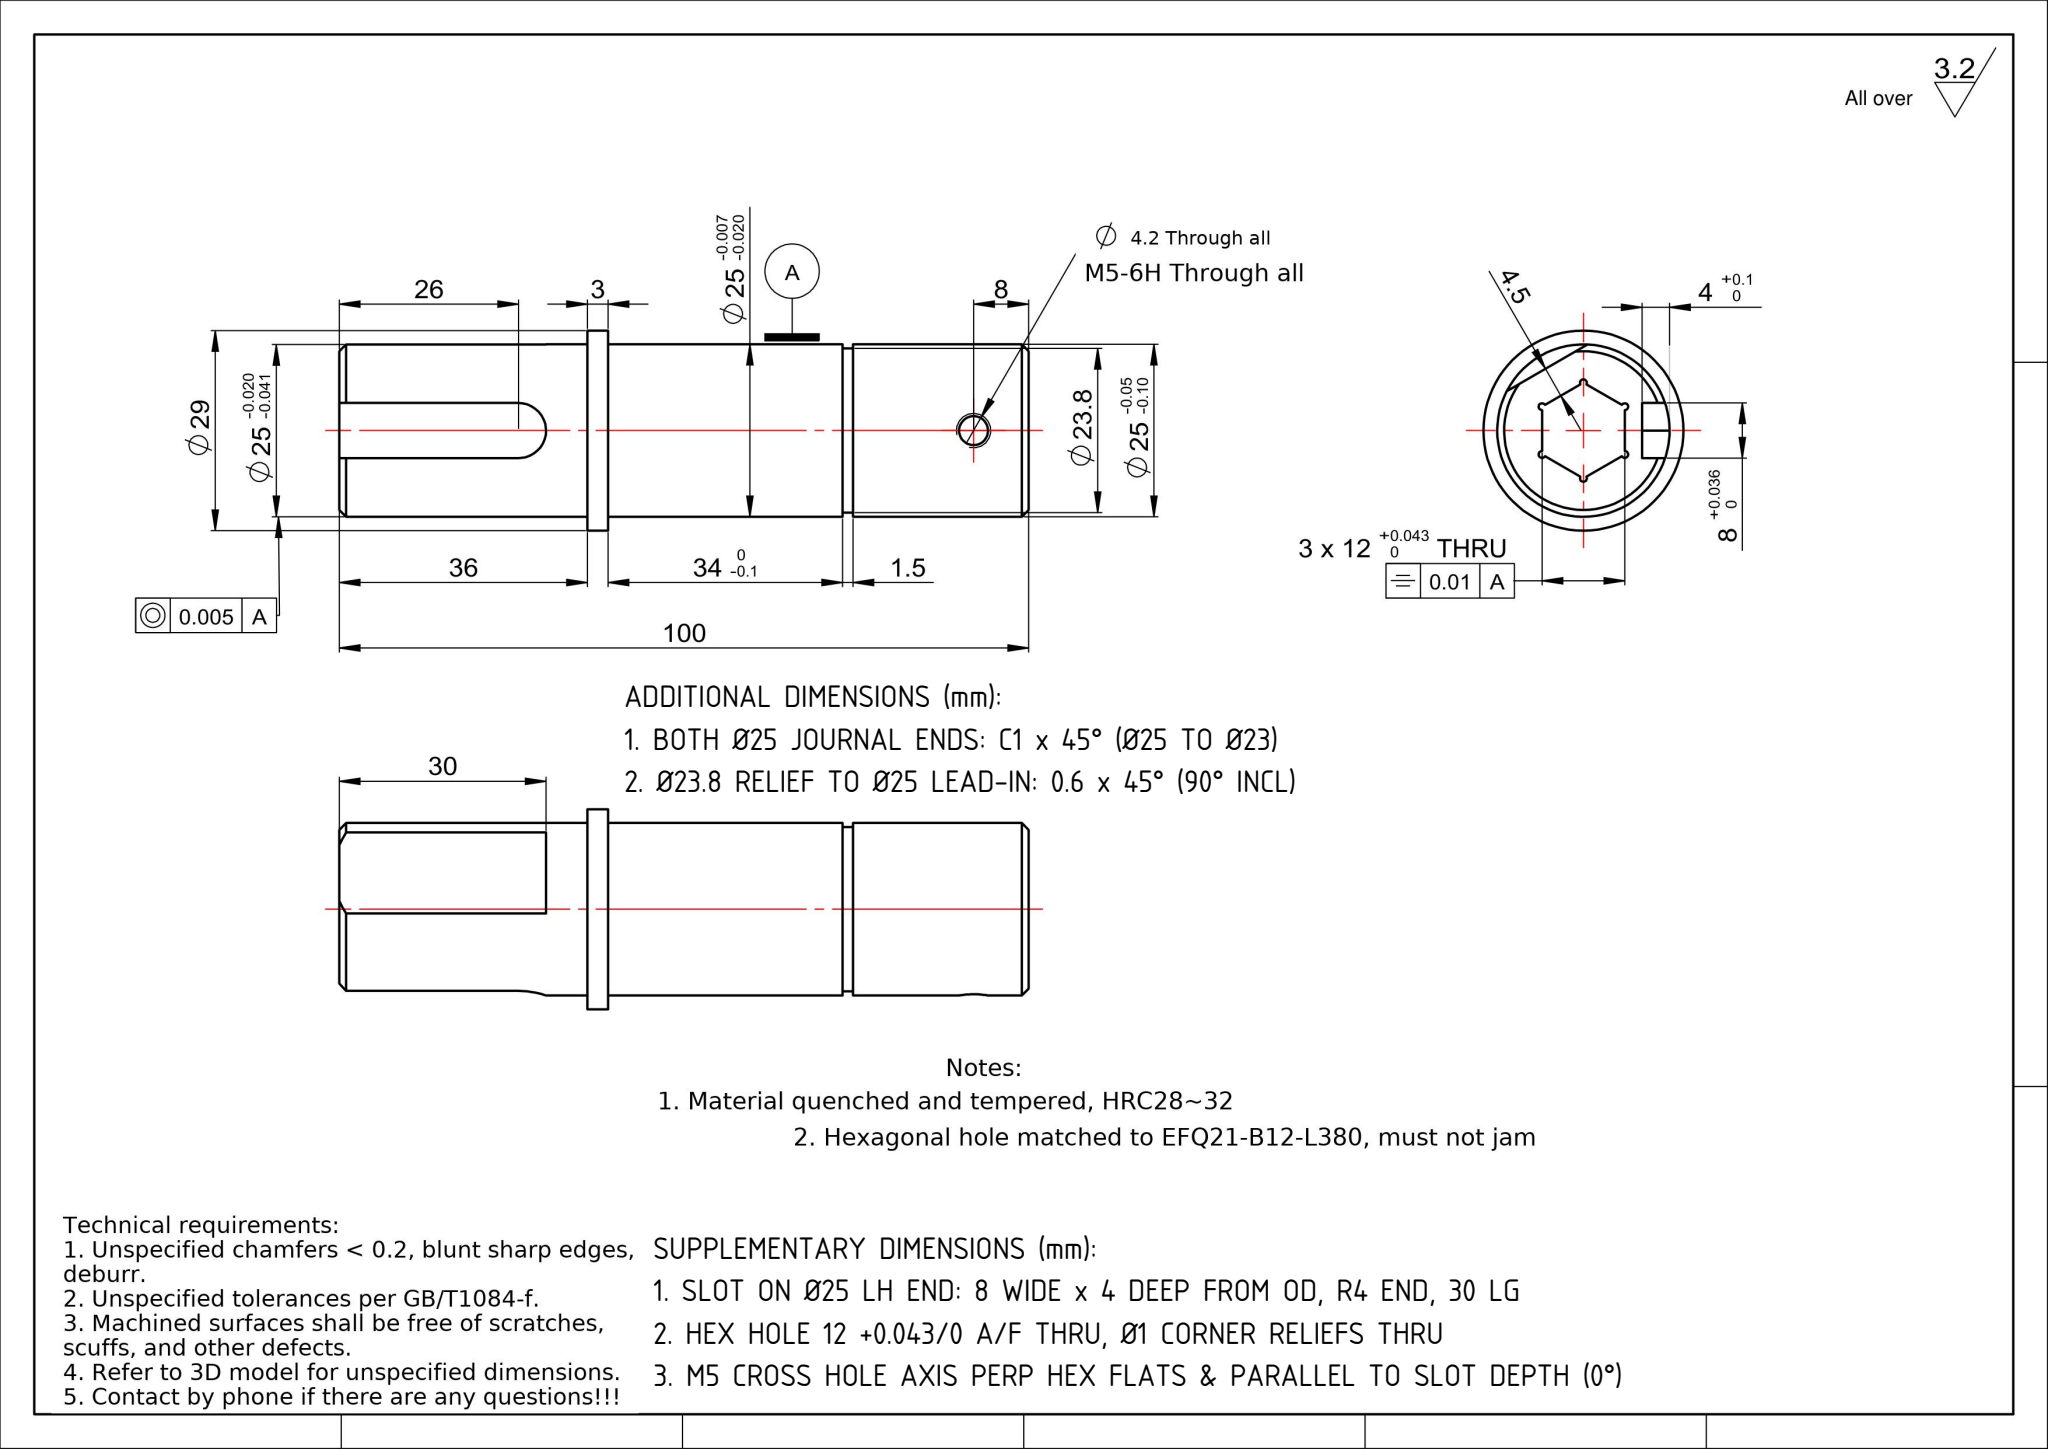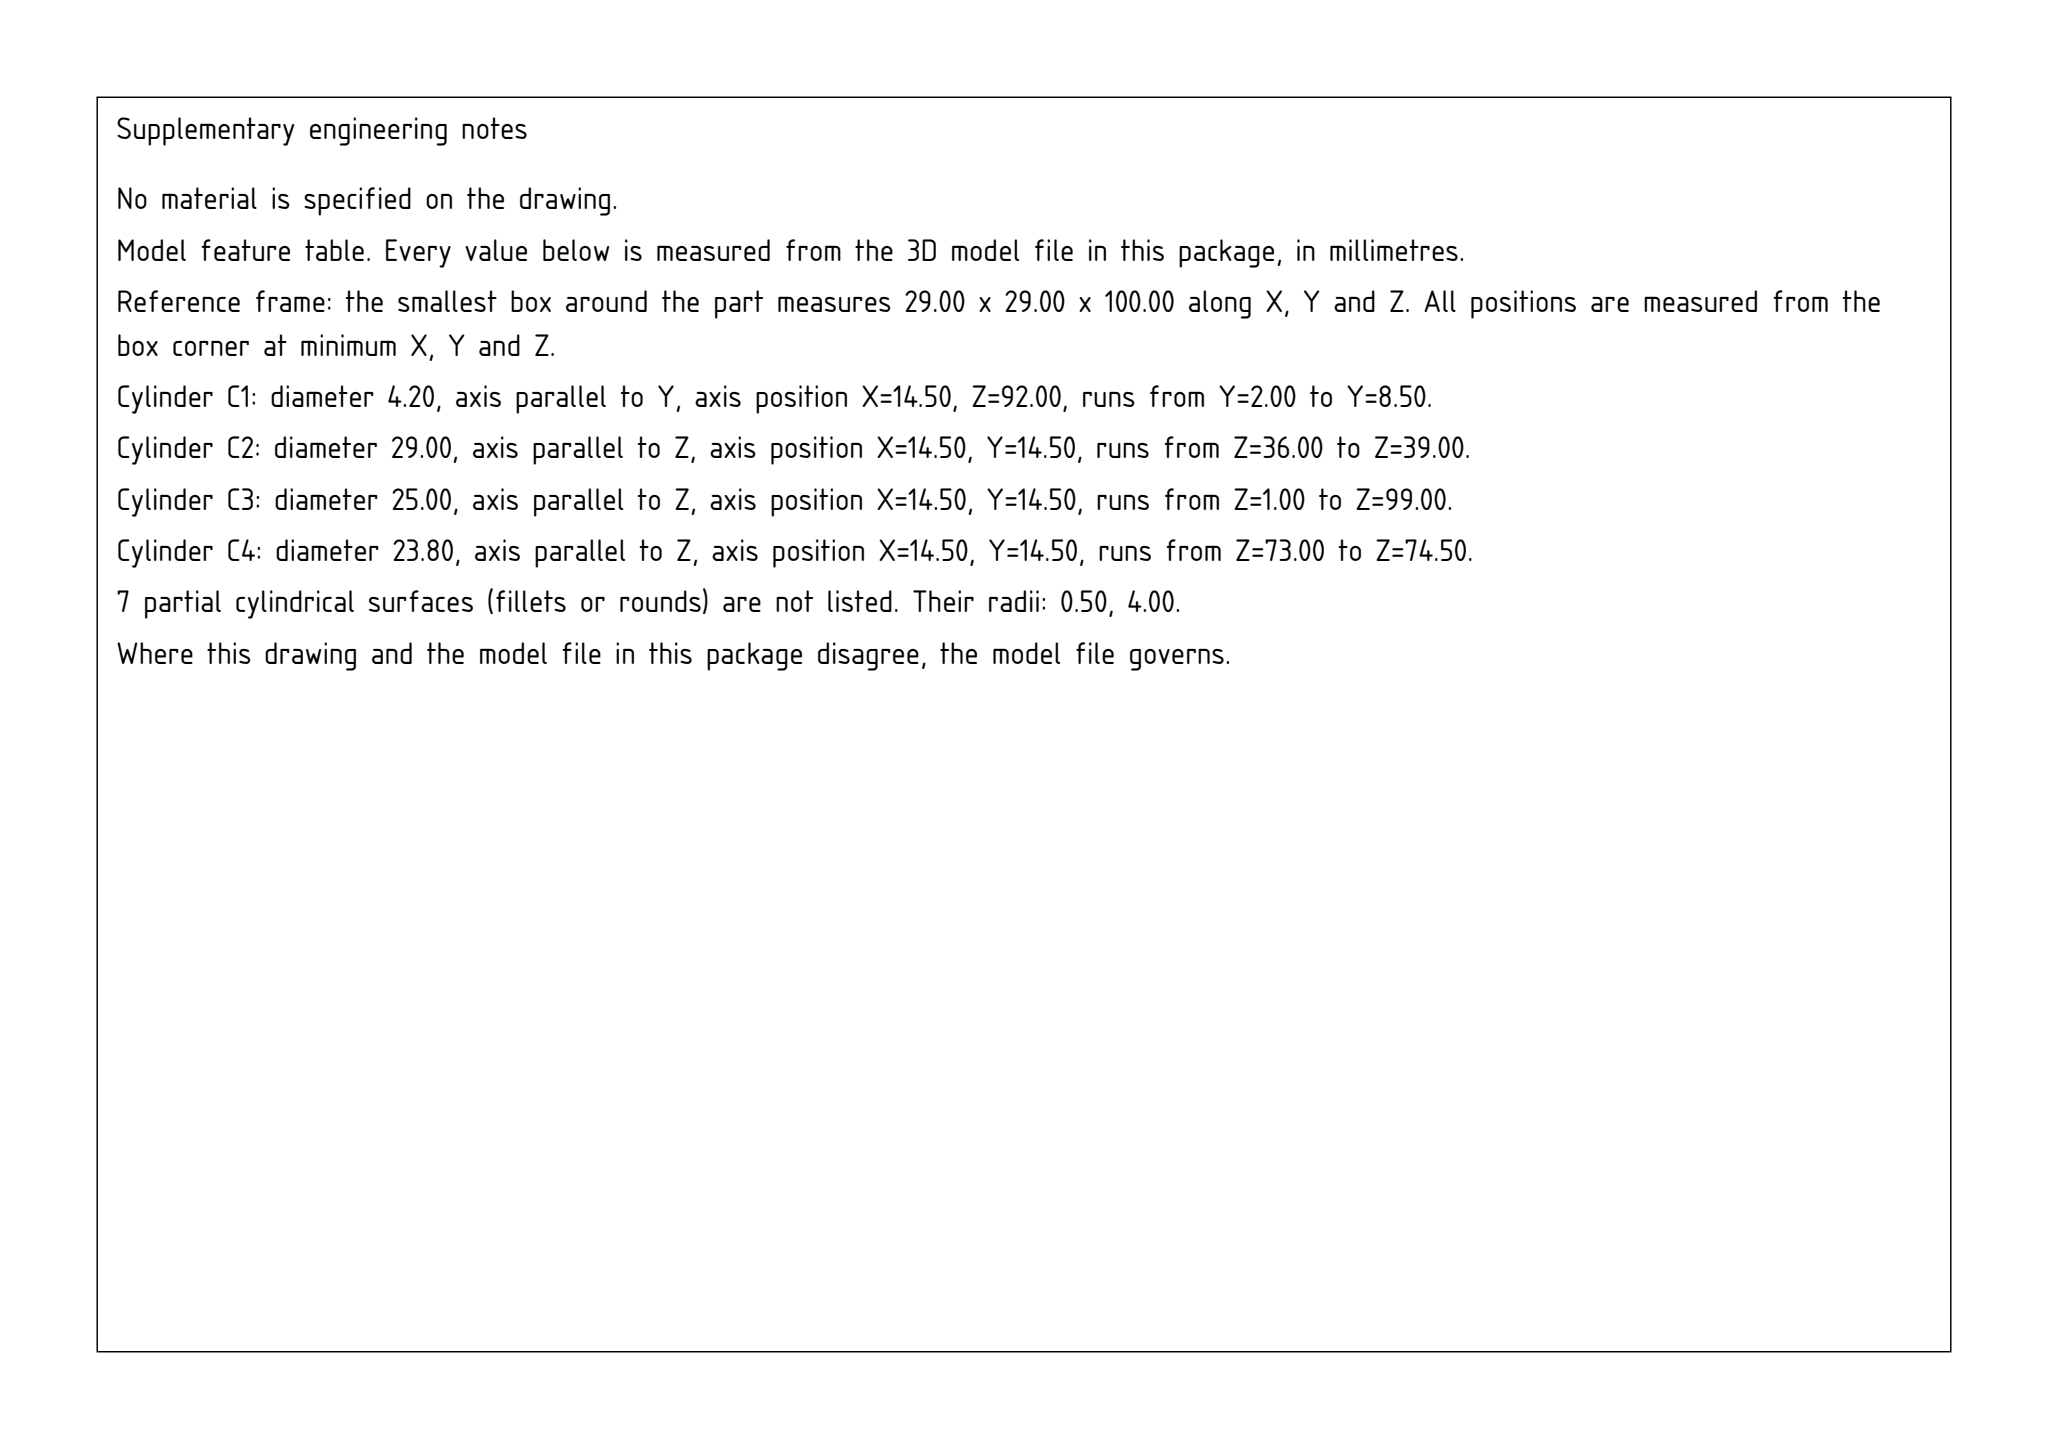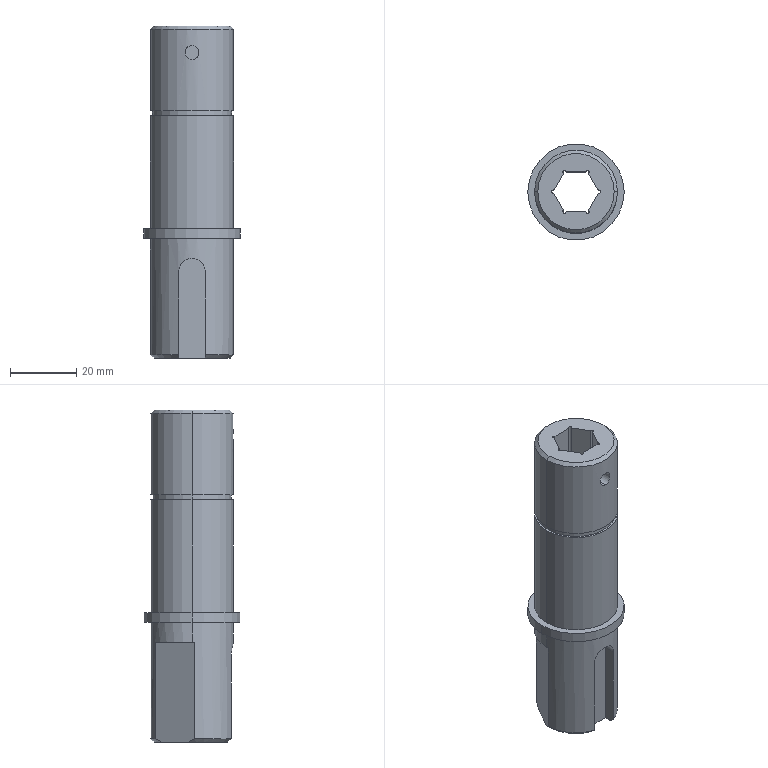Part | SolidWorks | mm | 1 solid | 45 faces | box 29 x 29 x 100 mm | volume 35152 mm3 | cylinder 23 | plane 17 | cone 5 | commonest cylinder face diameters 1 x9 25 x6 4.2 x2 23.8 x2 29 x2 8 x2